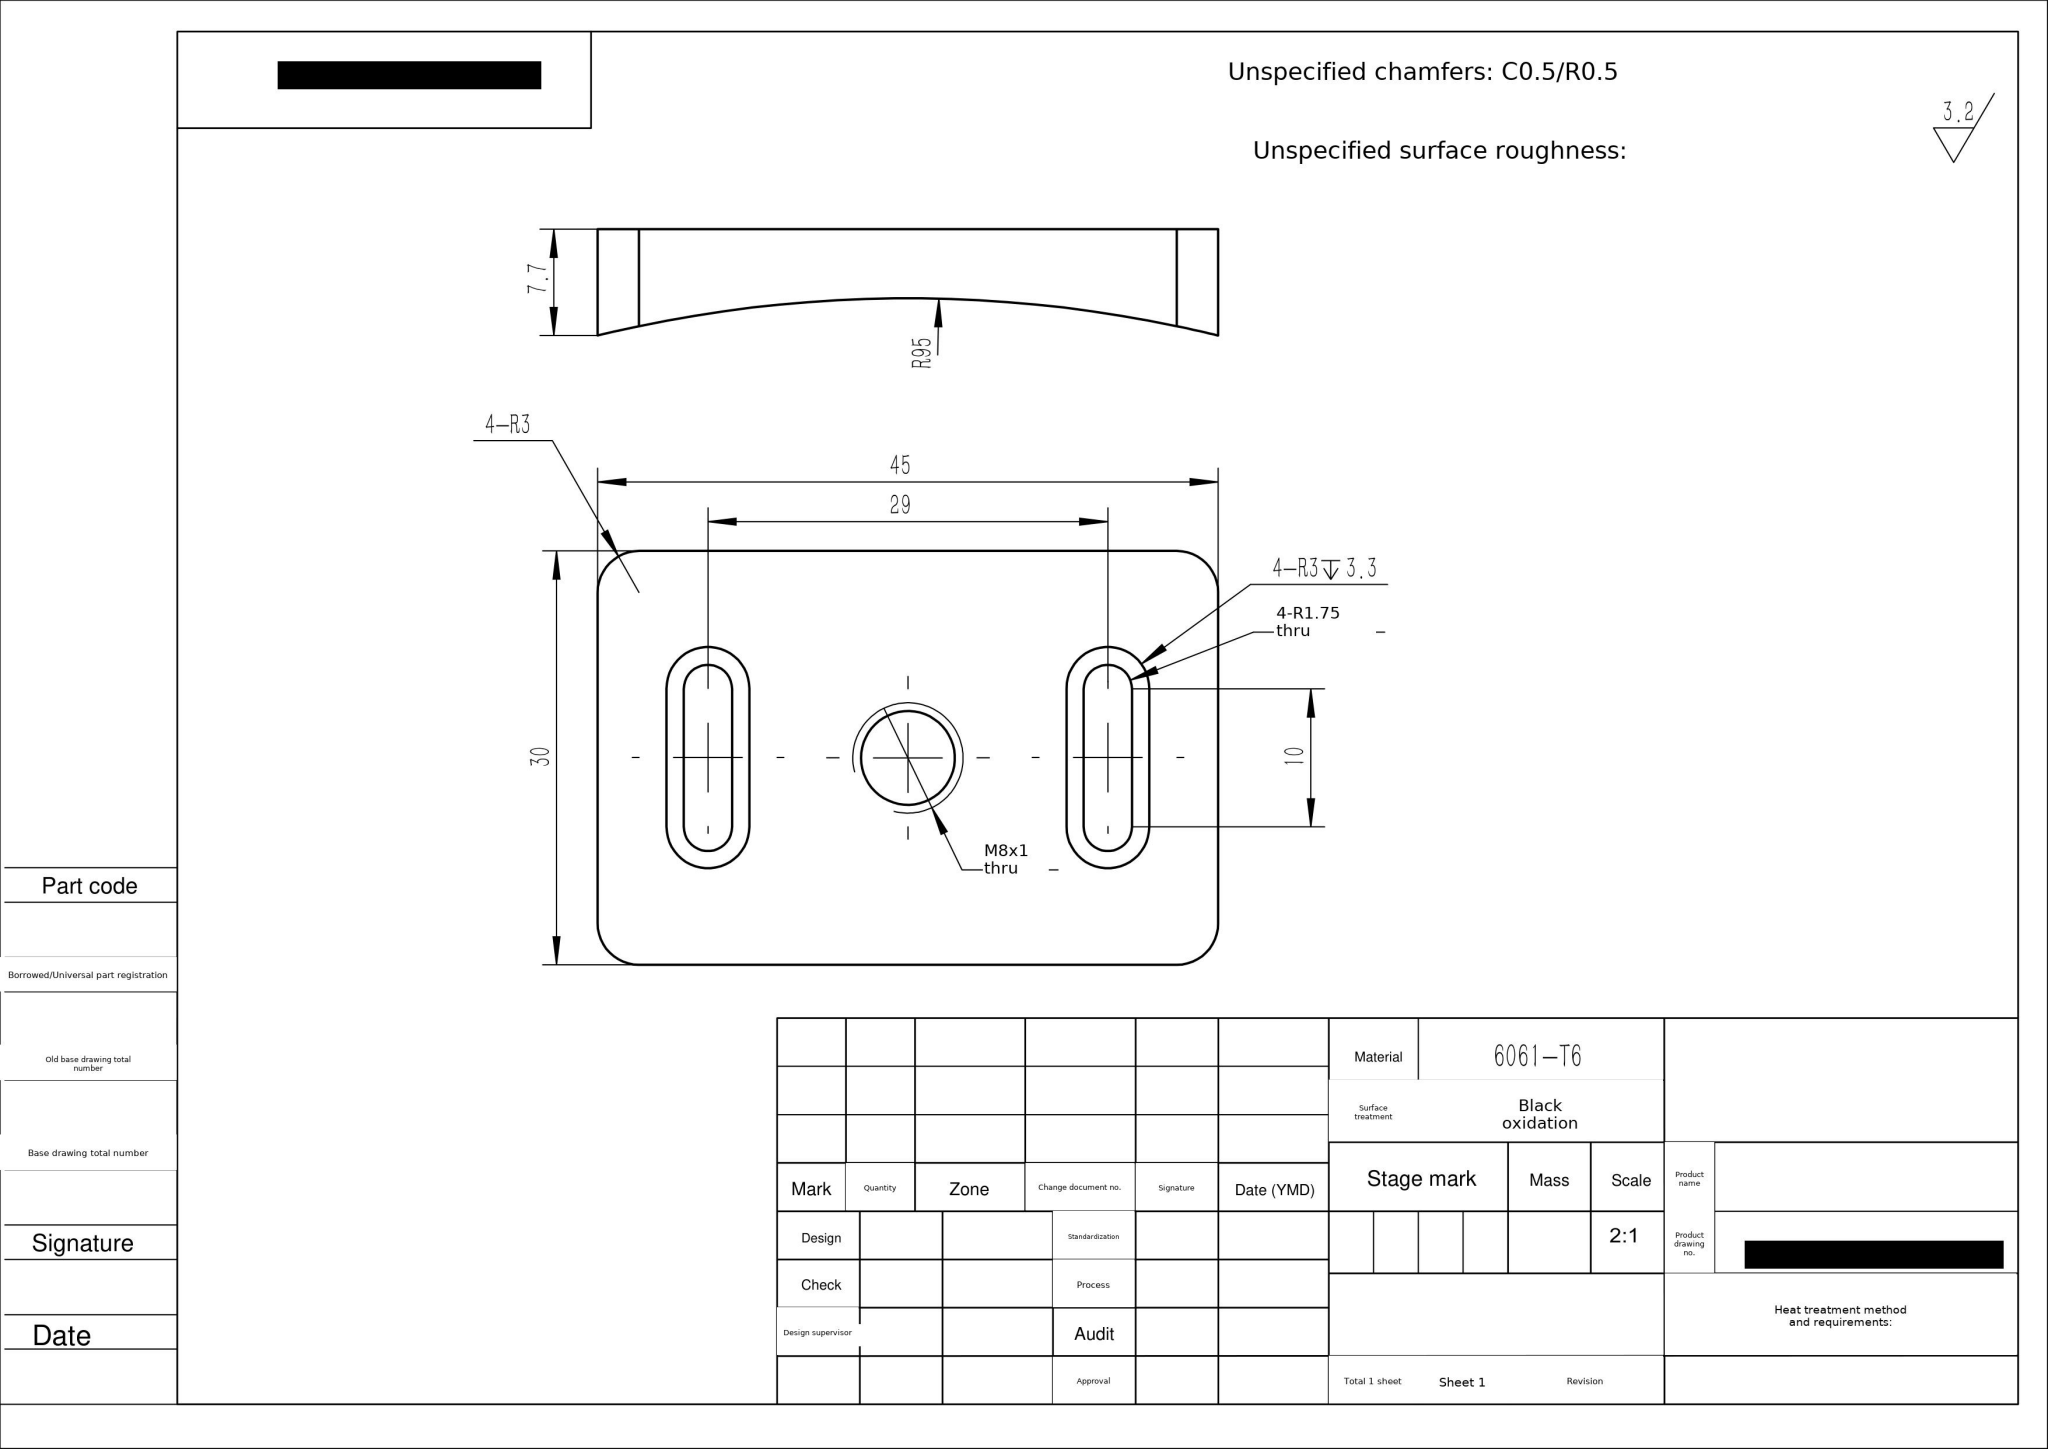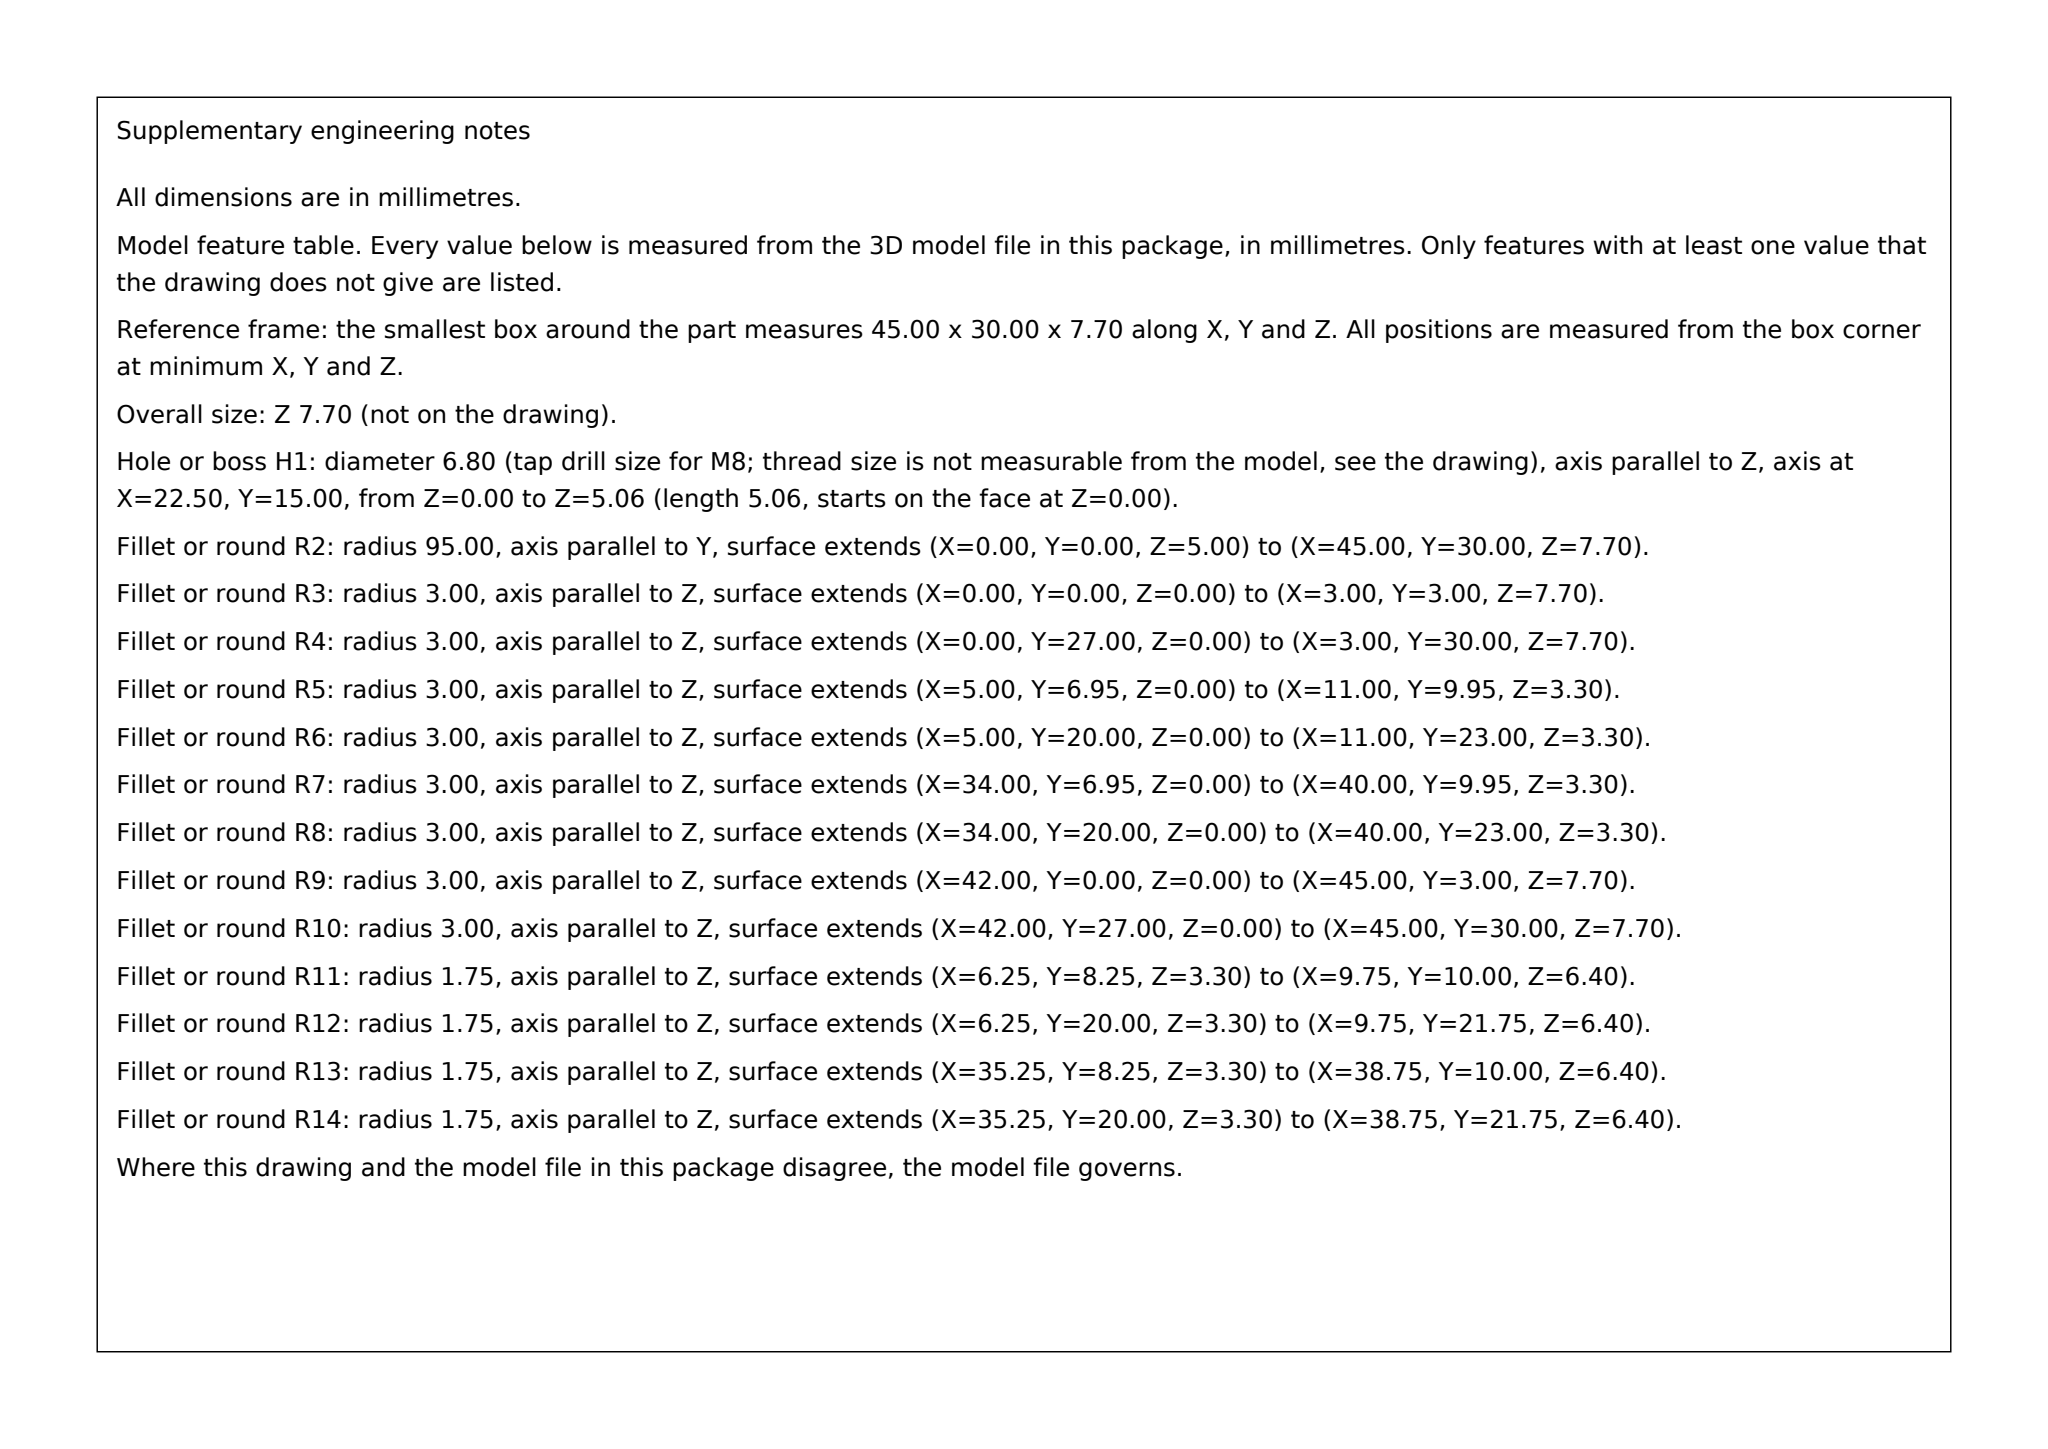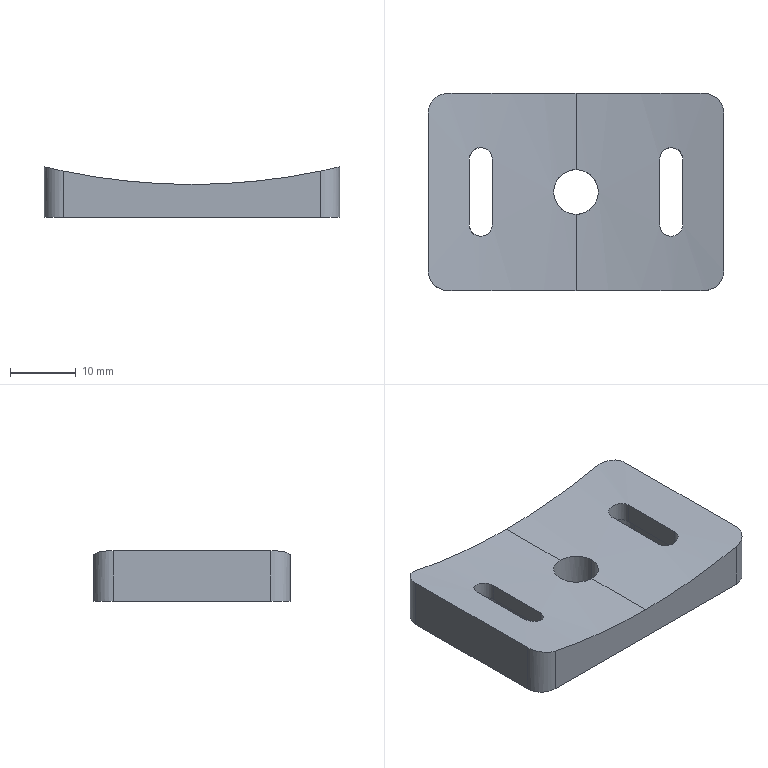Part | SolidWorks | mm | material 6061-T6 | 1 solid | 31 faces | box 45 x 30 x 7.7 mm | volume 6883 mm3 | cylinder 16 | plane 15 | commonest cylinder face diameters 6 x8 3.5 x4 6.8 x2 190 x2
build123d program:
from build123d import *

# Parameters (mm, degrees)
BOSS_EXTRUDE1_DEPTH = 30
FILLET1_R           = 3
M8_TAPPED_HOLE1_D   = 6.8
CUT_EXTRUDE1_DEPTH  = 39.283
CUT_EXTRUDE2_DEPTH  = 3.3


with BuildPart() as part:
    # Sketch1 → Boss-Extrude1 (new body)
    with BuildSketch(Plane(origin=(0, 0, 0), x_dir=(1, 0, 0), z_dir=(0, 1, 0))):
        with BuildLine():
            Line((-22.5, 92.297), (-22.5, 100))
            Line((-22.5, 100), (22.5, 100))
            Line((22.5, 100), (22.5, 92.297))
            ThreePointArc((22.5, 92.297), (0, 95), (-22.5, 92.297))
        make_face()
    extrude(amount=BOSS_EXTRUDE1_DEPTH)

    # Fillet1
    fillet1_edges = [part.edges().sort_by_distance(p)[0] for p in [
        (22.5, 30, -96.149),
        (22.5, 0, -96.149),
        (-22.5, 0, -96.149),
        (-22.5, 30, -96.149),
    ]]
    fillet(fillet1_edges, radius=FILLET1_R)

    # M8 Tapped Hole1 (through all)
    with Locations(Plane(origin=(0, 0, -100), x_dir=(-1, 0, 0), z_dir=(0, 0, -1))):
        with Locations((0, 15)):
            Hole(M8_TAPPED_HOLE1_D / 2)

    # Sketch4 → Cut-Extrude1 (cut, through all)
    with BuildSketch(Plane(origin=(0, 0, -100), x_dir=(-1, 0, 0), z_dir=(0, 0, -1))):
        with BuildLine():
            Line((-12.75, 20), (-12.75, 10))
            ThreePointArc((-12.75, 10), (-14.5, 8.25), (-16.25, 10))
            Line((-16.25, 10), (-16.25, 20))
            ThreePointArc((-16.25, 20), (-14.5, 21.75), (-12.75, 20))
        make_face()
        with BuildLine():
            Line((16.25, 20), (16.25, 10))
            ThreePointArc((16.25, 10), (14.5, 8.25), (12.75, 10))
            Line((12.75, 10), (12.75, 20))
            ThreePointArc((12.75, 20), (14.5, 21.75), (16.25, 20))
        make_face()
    extrude(amount=-CUT_EXTRUDE1_DEPTH, mode=Mode.SUBTRACT)

    # Sketch5 → Cut-Extrude2 (cut)
    with BuildSketch(Plane(origin=(0, 0, -100), x_dir=(-1, 0, 0), z_dir=(0, 0, -1))):
        with BuildLine():
            Line((-11.5, 20), (-11.5, 9.95))
            ThreePointArc((-11.5, 9.95), (-14.5, 6.95), (-17.5, 9.95))
            Line((-17.5, 9.95), (-17.5, 20))
            ThreePointArc((-17.5, 20), (-14.5, 23), (-11.5, 20))
        make_face()
        with BuildLine():
            Line((17.5, 20), (17.5, 9.95))
            ThreePointArc((17.5, 9.95), (14.5, 6.95), (11.5, 9.95))
            Line((11.5, 9.95), (11.5, 20))
            ThreePointArc((11.5, 20), (14.5, 23), (17.5, 20))
        make_face()
    extrude(amount=-CUT_EXTRUDE2_DEPTH, mode=Mode.SUBTRACT)


solid = part.part